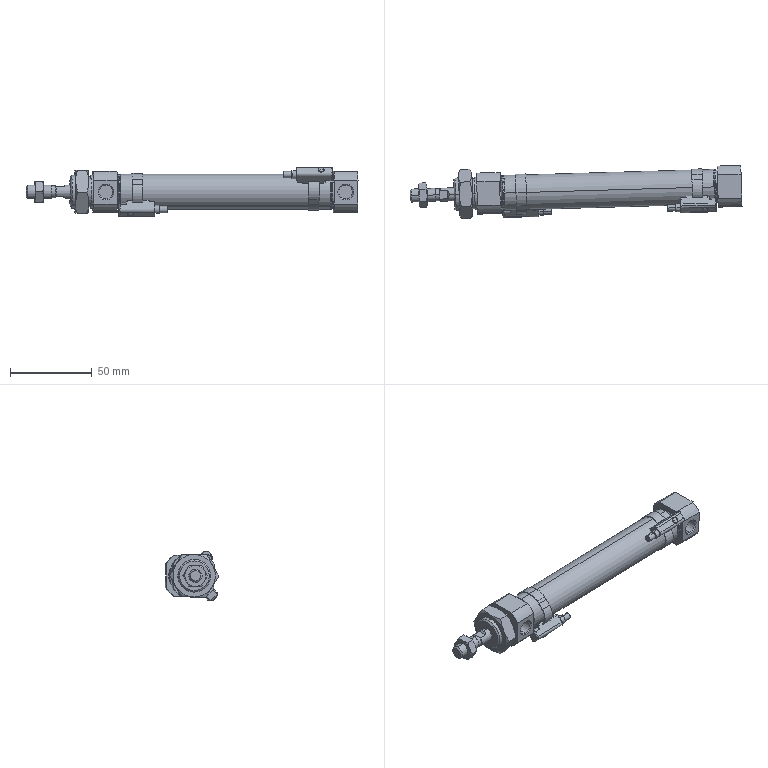Component | SolidWorks | MiniCylinderMF20x100SU_0_+_CS1-M-2-1 | 6 solids | 284 faces | volume 48247 mm3 | plane 130 | cylinder 96 | cone 42 | spline 16 | commonest cylinder face diameters 3.4 x14 21.4 x10 29 x8 16.4 x8 2 x8 20 x6 8 x6 8.566 x4 | material Standard Parts